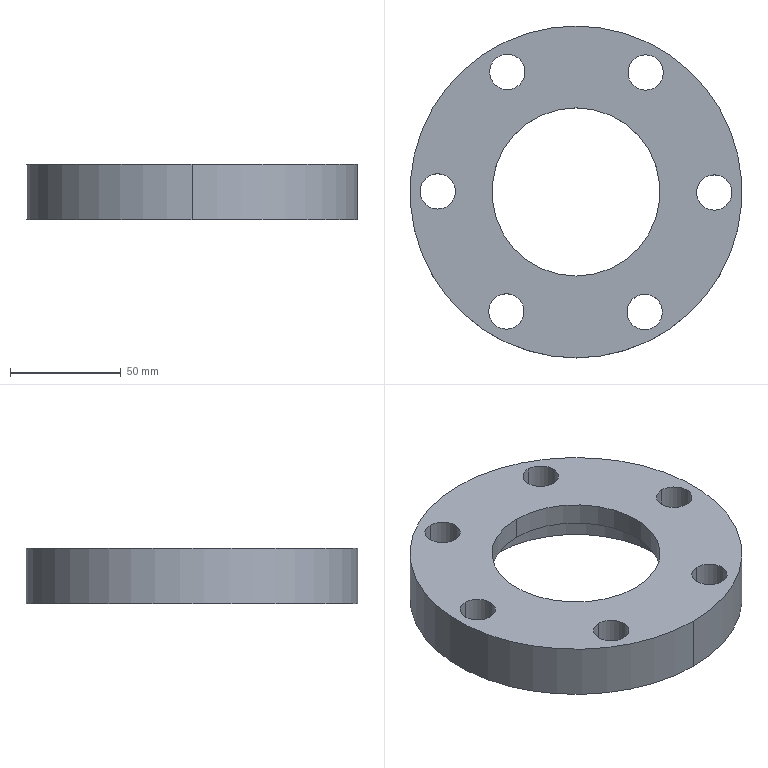Component | SolidWorks | Gland-1 | 1 solid | 21 faces | box 150 x 150 x 25 mm | volume 247272 mm3 | cylinder 18 | plane 3 | commonest cylinder face diameters 16 x12 100.5 x2 76 x2 150 x2
build123d program:
from build123d import *

# Parameters (mm, degrees)
SKETCH1_W                                  = 75
SKETCH1_H                                  = 25
F_16_0_16_DIAMETER_HOLE1_D                 = 16
M72_HEX_HEAD_BOLT_COUNTERBORE1_D           = 76
M72_HEX_HEAD_BOLT_COUNTERBORE1_CBORE_D     = 100.5
M72_HEX_HEAD_BOLT_COUNTERBORE1_CBORE_DEPTH = 15


with BuildPart() as part:
    # Sketch1 → Revolve1 (revolve)
    with BuildSketch(Plane.XZ, mode=Mode.PRIVATE) as revolve1_sk:
        with Locations((37.5, 12.5)):
            Rectangle(SKETCH1_W, SKETCH1_H)
    revolve(revolve1_sk.sketch.rotate(Axis((0, 0, 25), (0, 0, -1)), 180), axis=Axis((0, 0, 25), (0, 0, -1)))

    # 16.0 _16_ Diameter Hole1 (through all)
    with Locations(Plane.XY.offset(25)):
        with Locations((54.247, 31.035), (-54.001, 31.462), (-0.2468, -62.497), (-54.247, -31.035), (0.2468, 62.497), (54.001, -31.462)):
            Hole(F_16_0_16_DIAMETER_HOLE1_D / 2)

    # M72 Hex Head Bolt Counterbore1 (through all)
    with Locations(Plane(origin=(0, 0, 0), x_dir=(-1, 0, 0), z_dir=(0, 0, -1))):
        with Locations((0, 0)):
            CounterBoreHole(M72_HEX_HEAD_BOLT_COUNTERBORE1_D / 2, M72_HEX_HEAD_BOLT_COUNTERBORE1_CBORE_D / 2, M72_HEX_HEAD_BOLT_COUNTERBORE1_CBORE_DEPTH)


solid = part.part

# Placed as in the assembly
solid = solid.moved(Location((-505.158, 870.769, 814.663), (0, 0, 90)))
STEP:
#1=CARTESIAN_POINT('',(-19.888,36.261,32.664));
#2=VERTEX_POINT('',#1);
#3=CARTESIAN_POINT('',(-19.888,32.304,32.664));
#4=VERTEX_POINT('',#3);
#5=CARTESIAN_POINT('',(-19.888,34.282,32.664));
#6=DIRECTION('',(0.,0.,-1.));
#7=DIRECTION('',(0.,-1.,0.));
#8=AXIS2_PLACEMENT_3D('',#5,#6,#7);
#9=CIRCLE('',#8,1.978);
#10=EDGE_CURVE('',#2,#4,#9,.T.);
#11=ORIENTED_EDGE('',*,*,#10,.F.);
#12=CARTESIAN_POINT('',(-19.888,36.261,32.073));
#13=VERTEX_POINT('',#12);
#14=CARTESIAN_POINT('',(-19.888,36.261,32.073));
#15=DIRECTION('',(0.,0.,-1.));
#16=VECTOR('',#15,39.37);
#17=LINE('',#14,#16);
#18=EDGE_CURVE('',#2,#13,#17,.T.);
#19=ORIENTED_EDGE('',*,*,#18,.T.);
#20=CARTESIAN_POINT('',(-19.888,32.304,32.073));
#21=VERTEX_POINT('',#20);
#22=CARTESIAN_POINT('',(-19.888,34.282,32.073));
#23=DIRECTION('',(0.,0.,-1.));
#24=DIRECTION('',(0.,-1.,0.));
#25=AXIS2_PLACEMENT_3D('',#22,#23,#24);
#26=CIRCLE('',#25,1.978);
#27=EDGE_CURVE('',#13,#21,#26,.T.);
#28=ORIENTED_EDGE('',*,*,#27,.T.);
#29=CARTESIAN_POINT('',(-19.888,32.304,32.073));
#30=DIRECTION('',(0.,0.,-1.));
#31=VECTOR('',#30,39.37);
#32=LINE('',#29,#31);
#33=EDGE_CURVE('',#4,#21,#32,.T.);
#34=ORIENTED_EDGE('',*,*,#33,.F.);
#35=EDGE_LOOP('',(#11,#19,#28,#34));
#36=FACE_OUTER_BOUND('',#35,.T.);
#37=CARTESIAN_POINT('',(-19.888,34.282,32.073));
#38=DIRECTION('',(0.,0.,-1.));
#39=DIRECTION('',(0.,-1.,0.));
#40=AXIS2_PLACEMENT_3D('',#37,#38,#39);
#41=CYLINDRICAL_SURFACE('',#40,1.978);
#42=ADVANCED_FACE('',(#36),#41,.F.);
#43=CARTESIAN_POINT('',(-19.888,35.778,33.058));
#44=VERTEX_POINT('',#43);
#45=CARTESIAN_POINT('',(-19.888,32.786,33.058));
#46=VERTEX_POINT('',#45);
#47=CARTESIAN_POINT('',(-19.888,34.282,33.058));
#48=DIRECTION('',(0.,0.,-1.));
#49=DIRECTION('',(0.,-1.,0.));
#50=AXIS2_PLACEMENT_3D('',#47,#48,#49);
#51=CIRCLE('',#50,1.496);
#52=EDGE_CURVE('',#44,#46,#51,.T.);
#53=ORIENTED_EDGE('',*,*,#52,.F.);
#54=CARTESIAN_POINT('',(-19.888,35.778,32.664));
#55=VERTEX_POINT('',#54);
#56=CARTESIAN_POINT('',(-19.888,35.778,32.073));
#57=DIRECTION('',(0.,0.,-1.));
#58=VECTOR('',#57,39.37);
#59=LINE('',#56,#58);
#60=EDGE_CURVE('',#44,#55,#59,.T.);
#61=ORIENTED_EDGE('',*,*,#60,.T.);
#62=CARTESIAN_POINT('',(-19.888,32.786,32.664));
#63=VERTEX_POINT('',#62);
#64=CARTESIAN_POINT('',(-19.888,34.282,32.664));
#65=DIRECTION('',(0.,0.,-1.));
#66=DIRECTION('',(0.,-1.,0.));
#67=AXIS2_PLACEMENT_3D('',#64,#65,#66);
#68=CIRCLE('',#67,1.496);
#69=EDGE_CURVE('',#55,#63,#68,.T.);
#70=ORIENTED_EDGE('',*,*,#69,.T.);
#71=CARTESIAN_POINT('',(-19.888,32.786,32.073));
#72=DIRECTION('',(0.,0.,-1.));
#73=VECTOR('',#72,39.37);
#74=LINE('',#71,#73);
#75=EDGE_CURVE('',#46,#63,#74,.T.);
#76=ORIENTED_EDGE('',*,*,#75,.F.);
#77=EDGE_LOOP('',(#53,#61,#70,#76));
#78=FACE_OUTER_BOUND('',#77,.T.);
#79=CARTESIAN_POINT('',(-19.888,34.282,32.073));
#80=DIRECTION('',(0.,0.,-1.));
#81=DIRECTION('',(0.,-1.,0.));
#82=AXIS2_PLACEMENT_3D('',#79,#80,#81);
#83=CYLINDRICAL_SURFACE('',#82,1.496);
#84=ADVANCED_FACE('',(#78),#83,.F.);
#85=CARTESIAN_POINT('',(-21.11,36.103,32.073));
#86=VERTEX_POINT('',#85);
#87=CARTESIAN_POINT('',(-21.11,36.733,32.073));
#88=VERTEX_POINT('',#87);
#89=CARTESIAN_POINT('',(-21.11,36.418,32.073));
#90=DIRECTION('',(0.,0.,1.));
#91=DIRECTION('',(0.,1.,0.));
#92=AXIS2_PLACEMENT_3D('',#89,#90,#91);
#93=CIRCLE('',#92,0.315);
#94=EDGE_CURVE('',#86,#88,#93,.T.);
#95=ORIENTED_EDGE('',*,*,#94,.F.);
#96=CARTESIAN_POINT('',(-21.11,36.103,33.058));
#97=VERTEX_POINT('',#96);
#98=CARTESIAN_POINT('',(-21.11,36.103,33.058));
#99=DIRECTION('',(0.,0.,1.));
#100=VECTOR('',#99,39.37);
#101=LINE('',#98,#100);
#102=EDGE_CURVE('',#86,#97,#101,.T.);
#103=ORIENTED_EDGE('',*,*,#102,.T.);
#104=CARTESIAN_POINT('',(-21.11,36.733,33.058));
#105=VERTEX_POINT('',#104);
#106=CARTESIAN_POINT('',(-21.11,36.418,33.058));
#107=DIRECTION('',(0.,0.,1.));
#108=DIRECTION('',(0.,1.,0.));
#109=AXIS2_PLACEMENT_3D('',#106,#107,#108);
#110=CIRCLE('',#109,0.315);
#111=EDGE_CURVE('',#97,#105,#110,.T.);
#112=ORIENTED_EDGE('',*,*,#111,.T.);
#113=CARTESIAN_POINT('',(-21.11,36.733,33.058));
#114=DIRECTION('',(0.,0.,1.));
#115=VECTOR('',#114,39.37);
#116=LINE('',#113,#115);
#117=EDGE_CURVE('',#88,#105,#116,.T.);
#118=ORIENTED_EDGE('',*,*,#117,.F.);
#119=EDGE_LOOP('',(#95,#103,#112,#118));
#120=FACE_OUTER_BOUND('',#119,.T.);
#121=CARTESIAN_POINT('',(-21.11,36.418,33.058));
#122=DIRECTION('',(0.,0.,1.));
#123=DIRECTION('',(0.,1.,0.));
#124=AXIS2_PLACEMENT_3D('',#121,#122,#123);
#125=CYLINDRICAL_SURFACE('',#124,0.315);
#126=ADVANCED_FACE('',(#120),#125,.F.);
#127=CARTESIAN_POINT('',(-21.127,31.841,32.073));
#128=VERTEX_POINT('',#127);
#129=CARTESIAN_POINT('',(-21.127,32.471,32.073));
#130=VERTEX_POINT('',#129);
#131=CARTESIAN_POINT('',(-21.127,32.156,32.073));
#132=DIRECTION('',(0.,0.,1.));
#133=DIRECTION('',(0.,1.,0.));
#134=AXIS2_PLACEMENT_3D('',#131,#132,#133);
#135=CIRCLE('',#134,0.315);
#136=EDGE_CURVE('',#128,#130,#135,.T.);
#137=ORIENTED_EDGE('',*,*,#136,.F.);
#138=CARTESIAN_POINT('',(-21.127,31.841,33.058));
#139=VERTEX_POINT('',#138);
#140=CARTESIAN_POINT('',(-21.127,31.841,33.058));
#141=DIRECTION('',(0.,0.,1.));
#142=VECTOR('',#141,39.37);
#143=LINE('',#140,#142);
#144=EDGE_CURVE('',#128,#139,#143,.T.);
#145=ORIENTED_EDGE('',*,*,#144,.T.);
#146=CARTESIAN_POINT('',(-21.127,32.471,33.058));
#147=VERTEX_POINT('',#146);
#148=CARTESIAN_POINT('',(-21.127,32.156,33.058));
#149=DIRECTION('',(0.,0.,1.));
#150=DIRECTION('',(0.,1.,0.));
#151=AXIS2_PLACEMENT_3D('',#148,#149,#150);
#152=CIRCLE('',#151,0.315);
#153=EDGE_CURVE('',#139,#147,#152,.T.);
#154=ORIENTED_EDGE('',*,*,#153,.T.);
#155=CARTESIAN_POINT('',(-21.127,32.471,33.058));
#156=DIRECTION('',(0.,0.,1.));
#157=VECTOR('',#156,39.37);
#158=LINE('',#155,#157);
#159=EDGE_CURVE('',#130,#147,#158,.T.);
#160=ORIENTED_EDGE('',*,*,#159,.F.);
#161=EDGE_LOOP('',(#137,#145,#154,#160));
#162=FACE_OUTER_BOUND('',#161,.T.);
#163=CARTESIAN_POINT('',(-21.127,32.156,33.058));
#164=DIRECTION('',(0.,0.,1.));
#165=DIRECTION('',(0.,1.,0.));
#166=AXIS2_PLACEMENT_3D('',#163,#164,#165);
#167=CYLINDRICAL_SURFACE('',#166,0.315);
#168=ADVANCED_FACE('',(#162),#167,.F.);
#169=CARTESIAN_POINT('',(-17.428,33.958,32.073));
#170=VERTEX_POINT('',#169);
#171=CARTESIAN_POINT('',(-17.428,34.587,32.073));
#172=VERTEX_POINT('',#171);
#173=CARTESIAN_POINT('',(-17.428,34.273,32.073));
#174=DIRECTION('',(0.,0.,1.));
#175=DIRECTION('',(0.,1.,0.));
#176=AXIS2_PLACEMENT_3D('',#173,#174,#175);
#177=CIRCLE('',#176,0.315);
#178=EDGE_CURVE('',#170,#172,#177,.T.);
#179=ORIENTED_EDGE('',*,*,#178,.F.);
#180=CARTESIAN_POINT('',(-17.428,33.958,33.058));
#181=VERTEX_POINT('',#180);
#182=CARTESIAN_POINT('',(-17.428,33.958,33.058));
#183=DIRECTION('',(0.,0.,1.));
#184=VECTOR('',#183,39.37);
#185=LINE('',#182,#184);
#186=EDGE_CURVE('',#170,#181,#185,.T.);
#187=ORIENTED_EDGE('',*,*,#186,.T.);
#188=CARTESIAN_POINT('',(-17.428,34.587,33.058));
#189=VERTEX_POINT('',#188);
#190=CARTESIAN_POINT('',(-17.428,34.273,33.058));
#191=DIRECTION('',(0.,0.,1.));
#192=DIRECTION('',(0.,1.,0.));
#193=AXIS2_PLACEMENT_3D('',#190,#191,#192);
#194=CIRCLE('',#193,0.315);
#195=EDGE_CURVE('',#181,#189,#194,.T.);
#196=ORIENTED_EDGE('',*,*,#195,.T.);
#197=CARTESIAN_POINT('',(-17.428,34.587,33.058));
#198=DIRECTION('',(0.,0.,1.));
#199=VECTOR('',#198,39.37);
#200=LINE('',#197,#199);
#201=EDGE_CURVE('',#172,#189,#200,.T.);
#202=ORIENTED_EDGE('',*,*,#201,.F.);
#203=EDGE_LOOP('',(#179,#187,#196,#202));
#204=FACE_OUTER_BOUND('',#203,.T.);
#205=CARTESIAN_POINT('',(-17.428,34.273,33.058));
#206=DIRECTION('',(0.,0.,1.));
#207=DIRECTION('',(0.,1.,0.));
#208=AXIS2_PLACEMENT_3D('',#205,#206,#207);
#209=CYLINDRICAL_SURFACE('',#208,0.315);
#210=ADVANCED_FACE('',(#204),#209,.F.);
#211=CARTESIAN_POINT('',(-18.666,31.832,32.073));
#212=VERTEX_POINT('',#211);
#213=CARTESIAN_POINT('',(-18.666,32.461,32.073));
#214=VERTEX_POINT('',#213);
#215=CARTESIAN_POINT('',(-18.666,32.147,32.073));
#216=DIRECTION('',(0.,0.,1.));
#217=DIRECTION('',(0.,1.,0.));
#218=AXIS2_PLACEMENT_3D('',#215,#216,#217);
#219=CIRCLE('',#218,0.315);
#220=EDGE_CURVE('',#212,#214,#219,.T.);
#221=ORIENTED_EDGE('',*,*,#220,.F.);
#222=CARTESIAN_POINT('',(-18.666,31.832,33.058));
#223=VERTEX_POINT('',#222);
#224=CARTESIAN_POINT('',(-18.666,31.832,33.058));
#225=DIRECTION('',(0.,0.,1.));
#226=VECTOR('',#225,39.37);
#227=LINE('',#224,#226);
#228=EDGE_CURVE('',#212,#223,#227,.T.);
#229=ORIENTED_EDGE('',*,*,#228,.T.);
#230=CARTESIAN_POINT('',(-18.666,32.461,33.058));
#231=VERTEX_POINT('',#230);
#232=CARTESIAN_POINT('',(-18.666,32.147,33.058));
#233=DIRECTION('',(0.,0.,1.));
#234=DIRECTION('',(0.,1.,0.));
#235=AXIS2_PLACEMENT_3D('',#232,#233,#234);
#236=CIRCLE('',#235,0.315);
#237=EDGE_CURVE('',#223,#231,#236,.T.);
#238=ORIENTED_EDGE('',*,*,#237,.T.);
#239=CARTESIAN_POINT('',(-18.666,32.461,33.058));
#240=DIRECTION('',(0.,0.,1.));
#241=VECTOR('',#240,39.37);
#242=LINE('',#239,#241);
#243=EDGE_CURVE('',#214,#231,#242,.T.);
#244=ORIENTED_EDGE('',*,*,#243,.F.);
#245=EDGE_LOOP('',(#221,#229,#238,#244));
#246=FACE_OUTER_BOUND('',#245,.T.);
#247=CARTESIAN_POINT('',(-18.666,32.147,33.058));
#248=DIRECTION('',(0.,0.,1.));
#249=DIRECTION('',(0.,1.,0.));
#250=AXIS2_PLACEMENT_3D('',#247,#248,#249);
#251=CYLINDRICAL_SURFACE('',#250,0.315);
#252=ADVANCED_FACE('',(#246),#251,.F.);
#253=CARTESIAN_POINT('',(-22.349,33.977,32.073));
#254=VERTEX_POINT('',#253);
#255=CARTESIAN_POINT('',(-22.349,34.607,32.073));
#256=VERTEX_POINT('',#255);
#257=CARTESIAN_POINT('',(-22.349,34.292,32.073));
#258=DIRECTION('',(0.,0.,1.));
#259=DIRECTION('',(0.,1.,0.));
#260=AXIS2_PLACEMENT_3D('',#257,#258,#259);
#261=CIRCLE('',#260,0.315);
#262=EDGE_CURVE('',#254,#256,#261,.T.);
#263=ORIENTED_EDGE('',*,*,#262,.F.);
#264=CARTESIAN_POINT('',(-22.349,33.977,33.058));
#265=VERTEX_POINT('',#264);
#266=CARTESIAN_POINT('',(-22.349,33.977,33.058));
#267=DIRECTION('',(0.,0.,1.));
#268=VECTOR('',#267,39.37);
#269=LINE('',#266,#268);
#270=EDGE_CURVE('',#254,#265,#269,.T.);
#271=ORIENTED_EDGE('',*,*,#270,.T.);
#272=CARTESIAN_POINT('',(-22.349,34.607,33.058));
#273=VERTEX_POINT('',#272);
#274=CARTESIAN_POINT('',(-22.349,34.292,33.058));
#275=DIRECTION('',(0.,0.,1.));
#276=DIRECTION('',(0.,1.,0.));
#277=AXIS2_PLACEMENT_3D('',#274,#275,#276);
#278=CIRCLE('',#277,0.315);
#279=EDGE_CURVE('',#265,#273,#278,.T.);
#280=ORIENTED_EDGE('',*,*,#279,.T.);
#281=CARTESIAN_POINT('',(-22.349,34.607,33.058));
#282=DIRECTION('',(0.,0.,1.));
#283=VECTOR('',#282,39.37);
#284=LINE('',#281,#283);
#285=EDGE_CURVE('',#256,#273,#284,.T.);
#286=ORIENTED_EDGE('',*,*,#285,.F.);
#287=EDGE_LOOP('',(#263,#271,#280,#286));
#288=FACE_OUTER_BOUND('',#287,.T.);
#289=CARTESIAN_POINT('',(-22.349,34.292,33.058));
#290=DIRECTION('',(0.,0.,1.));
#291=DIRECTION('',(0.,1.,0.));
#292=AXIS2_PLACEMENT_3D('',#289,#290,#291);
#293=CYLINDRICAL_SURFACE('',#292,0.315);
#294=ADVANCED_FACE('',(#288),#293,.F.);
#295=CARTESIAN_POINT('',(-18.649,36.093,32.073));
#296=VERTEX_POINT('',#295);
#297=CARTESIAN_POINT('',(-18.649,36.723,32.073));
#298=VERTEX_POINT('',#297);
#299=CARTESIAN_POINT('',(-18.649,36.408,32.073));
#300=DIRECTION('',(0.,0.,1.));
#301=DIRECTION('',(0.,1.,0.));
#302=AXIS2_PLACEMENT_3D('',#299,#300,#301);
#303=CIRCLE('',#302,0.315);
#304=EDGE_CURVE('',#296,#298,#303,.T.);
#305=ORIENTED_EDGE('',*,*,#304,.F.);
#306=CARTESIAN_POINT('',(-18.649,36.093,33.058));
#307=VERTEX_POINT('',#306);
#308=CARTESIAN_POINT('',(-18.649,36.093,33.058));
#309=DIRECTION('',(0.,0.,1.));
#310=VECTOR('',#309,39.37);
#311=LINE('',#308,#310);
#312=EDGE_CURVE('',#296,#307,#311,.T.);
#313=ORIENTED_EDGE('',*,*,#312,.T.);
#314=CARTESIAN_POINT('',(-18.649,36.723,33.058));
#315=VERTEX_POINT('',#314);
#316=CARTESIAN_POINT('',(-18.649,36.408,33.058));
#317=DIRECTION('',(0.,0.,1.));
#318=DIRECTION('',(0.,1.,0.));
#319=AXIS2_PLACEMENT_3D('',#316,#317,#318);
#320=CIRCLE('',#319,0.315);
#321=EDGE_CURVE('',#307,#315,#320,.T.);
#322=ORIENTED_EDGE('',*,*,#321,.T.);
#323=CARTESIAN_POINT('',(-18.649,36.723,33.058));
#324=DIRECTION('',(0.,0.,1.));
#325=VECTOR('',#324,39.37);
#326=LINE('',#323,#325);
#327=EDGE_CURVE('',#298,#315,#326,.T.);
#328=ORIENTED_EDGE('',*,*,#327,.F.);
#329=EDGE_LOOP('',(#305,#313,#322,#328));
#330=FACE_OUTER_BOUND('',#329,.T.);
#331=CARTESIAN_POINT('',(-18.649,36.408,33.058));
#332=DIRECTION('',(0.,0.,1.));
#333=DIRECTION('',(0.,1.,0.));
#334=AXIS2_PLACEMENT_3D('',#331,#332,#333);
#335=CYLINDRICAL_SURFACE('',#334,0.315);
#336=ADVANCED_FACE('',(#330),#335,.F.);
#337=CARTESIAN_POINT('',(-19.888,31.329,33.058));
#338=VERTEX_POINT('',#337);
#339=CARTESIAN_POINT('',(-19.888,37.235,33.058));
#340=VERTEX_POINT('',#339);
#341=CARTESIAN_POINT('',(-19.888,34.282,33.058));
#342=DIRECTION('',(0.,0.,-1.));
#343=DIRECTION('',(0.,-1.,0.));
#344=AXIS2_PLACEMENT_3D('',#341,#342,#343);
#345=CIRCLE('',#344,2.953);
#346=EDGE_CURVE('',#338,#340,#345,.T.);
#347=ORIENTED_EDGE('',*,*,#346,.T.);
#348=CARTESIAN_POINT('',(-19.888,37.235,32.073));
#349=VERTEX_POINT('',#348);
#350=CARTESIAN_POINT('',(-19.888,37.235,33.058));
#351=DIRECTION('',(0.,0.,-1.));
#352=VECTOR('',#351,39.37);
#353=LINE('',#350,#352);
#354=EDGE_CURVE('',#340,#349,#353,.T.);
#355=ORIENTED_EDGE('',*,*,#354,.T.);
#356=CARTESIAN_POINT('',(-19.888,31.329,32.073));
#357=VERTEX_POINT('',#356);
#358=CARTESIAN_POINT('',(-19.888,34.282,32.073));
#359=DIRECTION('',(0.,0.,-1.));
#360=DIRECTION('',(0.,-1.,0.));
#361=AXIS2_PLACEMENT_3D('',#358,#359,#360);
#362=CIRCLE('',#361,2.953);
#363=EDGE_CURVE('',#357,#349,#362,.T.);
#364=ORIENTED_EDGE('',*,*,#363,.F.);
#365=CARTESIAN_POINT('',(-19.888,31.329,33.058));
#366=DIRECTION('',(0.,0.,-1.));
#367=VECTOR('',#366,39.37);
#368=LINE('',#365,#367);
#369=EDGE_CURVE('',#338,#357,#368,.T.);
#370=ORIENTED_EDGE('',*,*,#369,.F.);
#371=EDGE_LOOP('',(#347,#355,#364,#370));
#372=FACE_OUTER_BOUND('',#371,.T.);
#373=CARTESIAN_POINT('',(-19.888,34.282,33.058));
#374=DIRECTION('',(0.,0.,-1.));
#375=DIRECTION('',(0.,-1.,0.));
#376=AXIS2_PLACEMENT_3D('',#373,#374,#375);
#377=CYLINDRICAL_SURFACE('',#376,2.953);
#378=ADVANCED_FACE('',(#372),#377,.T.);
#379=CARTESIAN_POINT('',(-19.888,34.282,32.073));
#380=DIRECTION('',(0.,0.,-1.));
#381=DIRECTION('',(0.,-1.,0.));
#382=AXIS2_PLACEMENT_3D('',#379,#380,#381);
#383=CIRCLE('',#382,1.978);
#384=EDGE_CURVE('',#21,#13,#383,.T.);
#385=ORIENTED_EDGE('',*,*,#384,.F.);
#386=ORIENTED_EDGE('',*,*,#27,.F.);
#387=EDGE_LOOP('',(#385,#386));
#388=FACE_BOUND('',#387,.T.);
#389=CARTESIAN_POINT('',(-21.11,36.418,32.073));
#390=DIRECTION('',(0.,0.,1.));
#391=DIRECTION('',(0.,1.,0.));
#392=AXIS2_PLACEMENT_3D('',#389,#390,#391);
#393=CIRCLE('',#392,0.315);
#394=EDGE_CURVE('',#88,#86,#393,.T.);
#395=ORIENTED_EDGE('',*,*,#394,.T.);
#396=ORIENTED_EDGE('',*,*,#94,.T.);
#397=EDGE_LOOP('',(#395,#396));
#398=FACE_BOUND('',#397,.T.);
#399=CARTESIAN_POINT('',(-21.127,32.156,32.073));
#400=DIRECTION('',(0.,0.,1.));
#401=DIRECTION('',(0.,1.,0.));
#402=AXIS2_PLACEMENT_3D('',#399,#400,#401);
#403=CIRCLE('',#402,0.315);
#404=EDGE_CURVE('',#130,#128,#403,.T.);
#405=ORIENTED_EDGE('',*,*,#404,.T.);
#406=ORIENTED_EDGE('',*,*,#136,.T.);
#407=EDGE_LOOP('',(#405,#406));
#408=FACE_BOUND('',#407,.T.);
#409=ORIENTED_EDGE('',*,*,#363,.T.);
#410=CARTESIAN_POINT('',(-19.888,34.282,32.073));
#411=DIRECTION('',(0.,0.,-1.));
#412=DIRECTION('',(0.,-1.,0.));
#413=AXIS2_PLACEMENT_3D('',#410,#411,#412);
#414=CIRCLE('',#413,2.953);
#415=EDGE_CURVE('',#349,#357,#414,.T.);
#416=ORIENTED_EDGE('',*,*,#415,.T.);
#417=EDGE_LOOP('',(#409,#416));
#418=FACE_OUTER_BOUND('',#417,.T.);
#419=CARTESIAN_POINT('',(-18.649,36.408,32.073));
#420=DIRECTION('',(0.,0.,1.));
#421=DIRECTION('',(0.,1.,0.));
#422=AXIS2_PLACEMENT_3D('',#419,#420,#421);
#423=CIRCLE('',#422,0.315);
#424=EDGE_CURVE('',#298,#296,#423,.T.);
#425=ORIENTED_EDGE('',*,*,#424,.T.);
#426=ORIENTED_EDGE('',*,*,#304,.T.);
#427=EDGE_LOOP('',(#425,#426));
#428=FACE_BOUND('',#427,.T.);
#429=CARTESIAN_POINT('',(-22.349,34.292,32.073));
#430=DIRECTION('',(0.,0.,1.));
#431=DIRECTION('',(0.,1.,0.));
#432=AXIS2_PLACEMENT_3D('',#429,#430,#431);
#433=CIRCLE('',#432,0.315);
#434=EDGE_CURVE('',#256,#254,#433,.T.);
#435=ORIENTED_EDGE('',*,*,#434,.T.);
#436=ORIENTED_EDGE('',*,*,#262,.T.);
#437=EDGE_LOOP('',(#435,#436));
#438=FACE_BOUND('',#437,.T.);
#439=CARTESIAN_POINT('',(-18.666,32.147,32.073));
#440=DIRECTION('',(0.,0.,1.));
#441=DIRECTION('',(0.,1.,0.));
#442=AXIS2_PLACEMENT_3D('',#439,#440,#441);
#443=CIRCLE('',#442,0.315);
#444=EDGE_CURVE('',#214,#212,#443,.T.);
#445=ORIENTED_EDGE('',*,*,#444,.T.);
#446=ORIENTED_EDGE('',*,*,#220,.T.);
#447=EDGE_LOOP('',(#445,#446));
#448=FACE_BOUND('',#447,.T.);
#449=CARTESIAN_POINT('',(-17.428,34.273,32.073));
#450=DIRECTION('',(0.,0.,1.));
#451=DIRECTION('',(0.,1.,0.));
#452=AXIS2_PLACEMENT_3D('',#449,#450,#451);
#453=CIRCLE('',#452,0.315);
#454=EDGE_CURVE('',#172,#170,#453,.T.);
#455=ORIENTED_EDGE('',*,*,#454,.T.);
#456=ORIENTED_EDGE('',*,*,#178,.T.);
#457=EDGE_LOOP('',(#455,#456));
#458=FACE_BOUND('',#457,.T.);
#459=CARTESIAN_POINT('',(-19.888,34.282,32.073));
#460=DIRECTION('',(0.,0.,-1.));
#461=DIRECTION('',(0.,-1.,0.));
#462=AXIS2_PLACEMENT_3D('',#459,#460,#461);
#463=PLANE('',#462);
#464=ADVANCED_FACE('',(#388,#398,#408,#418,#428,#438,#448,#458),#463,.T.);
#465=ORIENTED_EDGE('',*,*,#354,.F.);
#466=CARTESIAN_POINT('',(-19.888,34.282,33.058));
#467=DIRECTION('',(0.,0.,-1.));
#468=DIRECTION('',(0.,-1.,0.));
#469=AXIS2_PLACEMENT_3D('',#466,#467,#468);
#470=CIRCLE('',#469,2.953);
#471=EDGE_CURVE('',#340,#338,#470,.T.);
#472=ORIENTED_EDGE('',*,*,#471,.T.);
#473=ORIENTED_EDGE('',*,*,#369,.T.);
#474=ORIENTED_EDGE('',*,*,#415,.F.);
#475=EDGE_LOOP('',(#465,#472,#473,#474));
#476=FACE_OUTER_BOUND('',#475,.T.);
#477=CARTESIAN_POINT('',(-19.888,34.282,33.058));
#478=DIRECTION('',(0.,0.,-1.));
#479=DIRECTION('',(0.,-1.,0.));
#480=AXIS2_PLACEMENT_3D('',#477,#478,#479);
#481=CYLINDRICAL_SURFACE('',#480,2.953);
#482=ADVANCED_FACE('',(#476),#481,.T.);
#483=CARTESIAN_POINT('',(-19.888,34.282,33.058));
#484=DIRECTION('',(0.,0.,-1.));
#485=DIRECTION('',(0.,-1.,0.));
#486=AXIS2_PLACEMENT_3D('',#483,#484,#485);
#487=CIRCLE('',#486,1.496);
#488=EDGE_CURVE('',#46,#44,#487,.T.);
#489=ORIENTED_EDGE('',*,*,#488,.T.);
#490=ORIENTED_EDGE('',*,*,#52,.T.);
#491=EDGE_LOOP('',(#489,#490));
#492=FACE_BOUND('',#491,.T.);
#493=CARTESIAN_POINT('',(-21.11,36.418,33.058));
#494=DIRECTION('',(0.,0.,1.));
#495=DIRECTION('',(0.,1.,0.));
#496=AXIS2_PLACEMENT_3D('',#493,#494,#495);
#497=CIRCLE('',#496,0.315);
#498=EDGE_CURVE('',#105,#97,#497,.T.);
#499=ORIENTED_EDGE('',*,*,#498,.F.);
#500=ORIENTED_EDGE('',*,*,#111,.F.);
#501=EDGE_LOOP('',(#499,#500));
#502=FACE_BOUND('',#501,.T.);
#503=CARTESIAN_POINT('',(-21.127,32.156,33.058));
#504=DIRECTION('',(0.,0.,1.));
#505=DIRECTION('',(0.,1.,0.));
#506=AXIS2_PLACEMENT_3D('',#503,#504,#505);
#507=CIRCLE('',#506,0.315);
#508=EDGE_CURVE('',#147,#139,#507,.T.);
#509=ORIENTED_EDGE('',*,*,#508,.F.);
#510=ORIENTED_EDGE('',*,*,#153,.F.);
#511=EDGE_LOOP('',(#509,#510));
#512=FACE_BOUND('',#511,.T.);
#513=CARTESIAN_POINT('',(-17.428,34.273,33.058));
#514=DIRECTION('',(0.,0.,1.));
#515=DIRECTION('',(0.,1.,0.));
#516=AXIS2_PLACEMENT_3D('',#513,#514,#515);
#517=CIRCLE('',#516,0.315);
#518=EDGE_CURVE('',#189,#181,#517,.T.);
#519=ORIENTED_EDGE('',*,*,#518,.F.);
#520=ORIENTED_EDGE('',*,*,#195,.F.);
#521=EDGE_LOOP('',(#519,#520));
#522=FACE_BOUND('',#521,.T.);
#523=CARTESIAN_POINT('',(-18.666,32.147,33.058));
#524=DIRECTION('',(0.,0.,1.));
#525=DIRECTION('',(0.,1.,0.));
#526=AXIS2_PLACEMENT_3D('',#523,#524,#525);
#527=CIRCLE('',#526,0.315);
#528=EDGE_CURVE('',#231,#223,#527,.T.);
#529=ORIENTED_EDGE('',*,*,#528,.F.);
#530=ORIENTED_EDGE('',*,*,#237,.F.);
#531=EDGE_LOOP('',(#529,#530));
#532=FACE_BOUND('',#531,.T.);
#533=CARTESIAN_POINT('',(-22.349,34.292,33.058));
#534=DIRECTION('',(0.,0.,1.));
#535=DIRECTION('',(0.,1.,0.));
#536=AXIS2_PLACEMENT_3D('',#533,#534,#535);
#537=CIRCLE('',#536,0.315);
#538=EDGE_CURVE('',#273,#265,#537,.T.);
#539=ORIENTED_EDGE('',*,*,#538,.F.);
#540=ORIENTED_EDGE('',*,*,#279,.F.);
#541=EDGE_LOOP('',(#539,#540));
#542=FACE_BOUND('',#541,.T.);
#543=CARTESIAN_POINT('',(-18.649,36.408,33.058));
#544=DIRECTION('',(0.,0.,1.));
#545=DIRECTION('',(0.,1.,0.));
#546=AXIS2_PLACEMENT_3D('',#543,#544,#545);
#547=CIRCLE('',#546,0.315);
#548=EDGE_CURVE('',#315,#307,#547,.T.);
#549=ORIENTED_EDGE('',*,*,#548,.F.);
#550=ORIENTED_EDGE('',*,*,#321,.F.);
#551=EDGE_LOOP('',(#549,#550));
#552=FACE_BOUND('',#551,.T.);
#553=ORIENTED_EDGE('',*,*,#346,.F.);
#554=ORIENTED_EDGE('',*,*,#471,.F.);
#555=EDGE_LOOP('',(#553,#554));
#556=FACE_OUTER_BOUND('',#555,.T.);
#557=CARTESIAN_POINT('',(-19.888,37.235,33.058));
#558=DIRECTION('',(0.,0.,1.));
#559=DIRECTION('',(0.,1.,0.));
#560=AXIS2_PLACEMENT_3D('',#557,#558,#559);
#561=PLANE('',#560);
#562=ADVANCED_FACE('',(#492,#502,#512,#522,#532,#542,#552,#556),#561,.T.);
#563=ORIENTED_EDGE('',*,*,#312,.F.);
#564=ORIENTED_EDGE('',*,*,#424,.F.);
#565=ORIENTED_EDGE('',*,*,#327,.T.);
#566=ORIENTED_EDGE('',*,*,#548,.T.);
#567=EDGE_LOOP('',(#563,#564,#565,#566));
#568=FACE_OUTER_BOUND('',#567,.T.);
#569=CARTESIAN_POINT('',(-18.649,36.408,33.058));
#570=DIRECTION('',(0.,0.,1.));
#571=DIRECTION('',(0.,1.,0.));
#572=AXIS2_PLACEMENT_3D('',#569,#570,#571);
#573=CYLINDRICAL_SURFACE('',#572,0.315);
#574=ADVANCED_FACE('',(#568),#573,.F.);
#575=ORIENTED_EDGE('',*,*,#270,.F.);
#576=ORIENTED_EDGE('',*,*,#434,.F.);
#577=ORIENTED_EDGE('',*,*,#285,.T.);
#578=ORIENTED_EDGE('',*,*,#538,.T.);
#579=EDGE_LOOP('',(#575,#576,#577,#578));
#580=FACE_OUTER_BOUND('',#579,.T.);
#581=CARTESIAN_POINT('',(-22.349,34.292,33.058));
#582=DIRECTION('',(0.,0.,1.));
#583=DIRECTION('',(0.,1.,0.));
#584=AXIS2_PLACEMENT_3D('',#581,#582,#583);
#585=CYLINDRICAL_SURFACE('',#584,0.315);
#586=ADVANCED_FACE('',(#580),#585,.F.);
#587=ORIENTED_EDGE('',*,*,#228,.F.);
#588=ORIENTED_EDGE('',*,*,#444,.F.);
#589=ORIENTED_EDGE('',*,*,#243,.T.);
#590=ORIENTED_EDGE('',*,*,#528,.T.);
#591=EDGE_LOOP('',(#587,#588,#589,#590));
#592=FACE_OUTER_BOUND('',#591,.T.);
#593=CARTESIAN_POINT('',(-18.666,32.147,33.058));
#594=DIRECTION('',(0.,0.,1.));
#595=DIRECTION('',(0.,1.,0.));
#596=AXIS2_PLACEMENT_3D('',#593,#594,#595);
#597=CYLINDRICAL_SURFACE('',#596,0.315);
#598=ADVANCED_FACE('',(#592),#597,.F.);
#599=ORIENTED_EDGE('',*,*,#186,.F.);
#600=ORIENTED_EDGE('',*,*,#454,.F.);
#601=ORIENTED_EDGE('',*,*,#201,.T.);
#602=ORIENTED_EDGE('',*,*,#518,.T.);
#603=EDGE_LOOP('',(#599,#600,#601,#602));
#604=FACE_OUTER_BOUND('',#603,.T.);
#605=CARTESIAN_POINT('',(-17.428,34.273,33.058));
#606=DIRECTION('',(0.,0.,1.));
#607=DIRECTION('',(0.,1.,0.));
#608=AXIS2_PLACEMENT_3D('',#605,#606,#607);
#609=CYLINDRICAL_SURFACE('',#608,0.315);
#610=ADVANCED_FACE('',(#604),#609,.F.);
#611=ORIENTED_EDGE('',*,*,#144,.F.);
#612=ORIENTED_EDGE('',*,*,#404,.F.);
#613=ORIENTED_EDGE('',*,*,#159,.T.);
#614=ORIENTED_EDGE('',*,*,#508,.T.);
#615=EDGE_LOOP('',(#611,#612,#613,#614));
#616=FACE_OUTER_BOUND('',#615,.T.);
#617=CARTESIAN_POINT('',(-21.127,32.156,33.058));
#618=DIRECTION('',(0.,0.,1.));
#619=DIRECTION('',(0.,1.,0.));
#620=AXIS2_PLACEMENT_3D('',#617,#618,#619);
#621=CYLINDRICAL_SURFACE('',#620,0.315);
#622=ADVANCED_FACE('',(#616),#621,.F.);
#623=ORIENTED_EDGE('',*,*,#102,.F.);
#624=ORIENTED_EDGE('',*,*,#394,.F.);
#625=ORIENTED_EDGE('',*,*,#117,.T.);
#626=ORIENTED_EDGE('',*,*,#498,.T.);
#627=EDGE_LOOP('',(#623,#624,#625,#626));
#628=FACE_OUTER_BOUND('',#627,.T.);
#629=CARTESIAN_POINT('',(-21.11,36.418,33.058));
#630=DIRECTION('',(0.,0.,1.));
#631=DIRECTION('',(0.,1.,0.));
#632=AXIS2_PLACEMENT_3D('',#629,#630,#631);
#633=CYLINDRICAL_SURFACE('',#632,0.315);
#634=ADVANCED_FACE('',(#628),#633,.F.);
#635=ORIENTED_EDGE('',*,*,#60,.F.);
#636=ORIENTED_EDGE('',*,*,#488,.F.);
#637=ORIENTED_EDGE('',*,*,#75,.T.);
#638=CARTESIAN_POINT('',(-19.888,34.282,32.664));
#639=DIRECTION('',(0.,0.,-1.));
#640=DIRECTION('',(0.,-1.,0.));
#641=AXIS2_PLACEMENT_3D('',#638,#639,#640);
#642=CIRCLE('',#641,1.496);
#643=EDGE_CURVE('',#63,#55,#642,.T.);
#644=ORIENTED_EDGE('',*,*,#643,.T.);
#645=EDGE_LOOP('',(#635,#636,#637,#644));
#646=FACE_OUTER_BOUND('',#645,.T.);
#647=CARTESIAN_POINT('',(-19.888,34.282,32.073));
#648=DIRECTION('',(0.,0.,-1.));
#649=DIRECTION('',(0.,-1.,0.));
#650=AXIS2_PLACEMENT_3D('',#647,#648,#649);
#651=CYLINDRICAL_SURFACE('',#650,1.496);
#652=ADVANCED_FACE('',(#646),#651,.F.);
#653=ORIENTED_EDGE('',*,*,#643,.F.);
#654=ORIENTED_EDGE('',*,*,#69,.F.);
#655=EDGE_LOOP('',(#653,#654));
#656=FACE_BOUND('',#655,.T.);
#657=CARTESIAN_POINT('',(-19.888,34.282,32.664));
#658=DIRECTION('',(0.,0.,-1.));
#659=DIRECTION('',(0.,-1.,0.));
#660=AXIS2_PLACEMENT_3D('',#657,#658,#659);
#661=CIRCLE('',#660,1.978);
#662=EDGE_CURVE('',#4,#2,#661,.T.);
#663=ORIENTED_EDGE('',*,*,#662,.T.);
#664=ORIENTED_EDGE('',*,*,#10,.T.);
#665=EDGE_LOOP('',(#663,#664));
#666=FACE_OUTER_BOUND('',#665,.T.);
#667=CARTESIAN_POINT('',(-19.888,35.778,32.664));
#668=DIRECTION('',(0.,0.,1.));
#669=DIRECTION('',(0.,1.,0.));
#670=AXIS2_PLACEMENT_3D('',#667,#668,#669);
#671=PLANE('',#670);
#672=ADVANCED_FACE('',(#656,#666),#671,.F.);
#673=ORIENTED_EDGE('',*,*,#18,.F.);
#674=ORIENTED_EDGE('',*,*,#662,.F.);
#675=ORIENTED_EDGE('',*,*,#33,.T.);
#676=ORIENTED_EDGE('',*,*,#384,.T.);
#677=EDGE_LOOP('',(#673,#674,#675,#676));
#678=FACE_OUTER_BOUND('',#677,.T.);
#679=CARTESIAN_POINT('',(-19.888,34.282,32.073));
#680=DIRECTION('',(0.,0.,-1.));
#681=DIRECTION('',(0.,-1.,0.));
#682=AXIS2_PLACEMENT_3D('',#679,#680,#681);
#683=CYLINDRICAL_SURFACE('',#682,1.978);
#684=ADVANCED_FACE('',(#678),#683,.F.);
#685=CLOSED_SHELL('',(#42,#84,#126,#168,#210,#252,#294,#336,#378,#464,#482,#562,#574,#586,#598,#610,#622,#634,#652,#672,#684));
#686=MANIFOLD_SOLID_BREP('',#685);
#687=CARTESIAN_POINT('',(0.,0.,0.));
#688=DIRECTION('',(0.,0.,1.));
#689=DIRECTION('',(1.,0.,0.));
#690=AXIS2_PLACEMENT_3D('',#687,#688,#689);
#691=(LENGTH_UNIT()NAMED_UNIT(*)SI_UNIT($,.METRE.));
#692=LENGTH_MEASURE_WITH_UNIT(LENGTH_MEASURE(0.0254),#691);
#693=DIMENSIONAL_EXPONENTS(1.,0.,0.,0.,0.,0.,0.);
#694=(CONVERSION_BASED_UNIT('',#692)LENGTH_UNIT()NAMED_UNIT(#693));
#695=UNCERTAINTY_MEASURE_WITH_UNIT(LENGTH_MEASURE(0.00001),#694,'','');
#696=(NAMED_UNIT(*)PLANE_ANGLE_UNIT()SI_UNIT($,.RADIAN.));
#697=(NAMED_UNIT(*)SI_UNIT($,.STERADIAN.)SOLID_ANGLE_UNIT());
#698=(GEOMETRIC_REPRESENTATION_CONTEXT(3)GLOBAL_UNCERTAINTY_ASSIGNED_CONTEXT((#695))GLOBAL_UNIT_ASSIGNED_CONTEXT((#694,#696,#697))REPRESENTATION_CONTEXT('',''));
#699=ADVANCED_BREP_SHAPE_REPRESENTATION('',(#686,#690),#698);
#700=COLOUR_RGB('',0.7922,0.8196,0.9333);
#701=FILL_AREA_STYLE_COLOUR('',#700);
#702=FILL_AREA_STYLE('',(#701));
#703=SURFACE_STYLE_FILL_AREA(#702);
#704=SURFACE_SIDE_STYLE('',(#703));
#705=SURFACE_STYLE_USAGE(.BOTH.,#704);
#706=PRESENTATION_STYLE_ASSIGNMENT((#705));
#707=STYLED_ITEM('',(#706),#686);
#708=PRESENTATION_LAYER_ASSIGNMENT('','',(#707));
#709=(LENGTH_UNIT()NAMED_UNIT(*)SI_UNIT($,.METRE.));
#710=LENGTH_MEASURE_WITH_UNIT(LENGTH_MEASURE(0.0254),#709);
#711=DIMENSIONAL_EXPONENTS(1.,0.,0.,0.,0.,0.,0.);
#712=(CONVERSION_BASED_UNIT('',#710)LENGTH_UNIT()NAMED_UNIT(#711));
#713=UNCERTAINTY_MEASURE_WITH_UNIT(LENGTH_MEASURE(0.00001),#712,'','');
#714=(NAMED_UNIT(*)PLANE_ANGLE_UNIT()SI_UNIT($,.RADIAN.));
#715=(NAMED_UNIT(*)SI_UNIT($,.STERADIAN.)SOLID_ANGLE_UNIT());
#716=(GEOMETRIC_REPRESENTATION_CONTEXT(3)GLOBAL_UNCERTAINTY_ASSIGNED_CONTEXT((#713))GLOBAL_UNIT_ASSIGNED_CONTEXT((#712,#714,#715))REPRESENTATION_CONTEXT('',''));
#717=MECHANICAL_DESIGN_GEOMETRIC_PRESENTATION_REPRESENTATION('',(#707),#716);